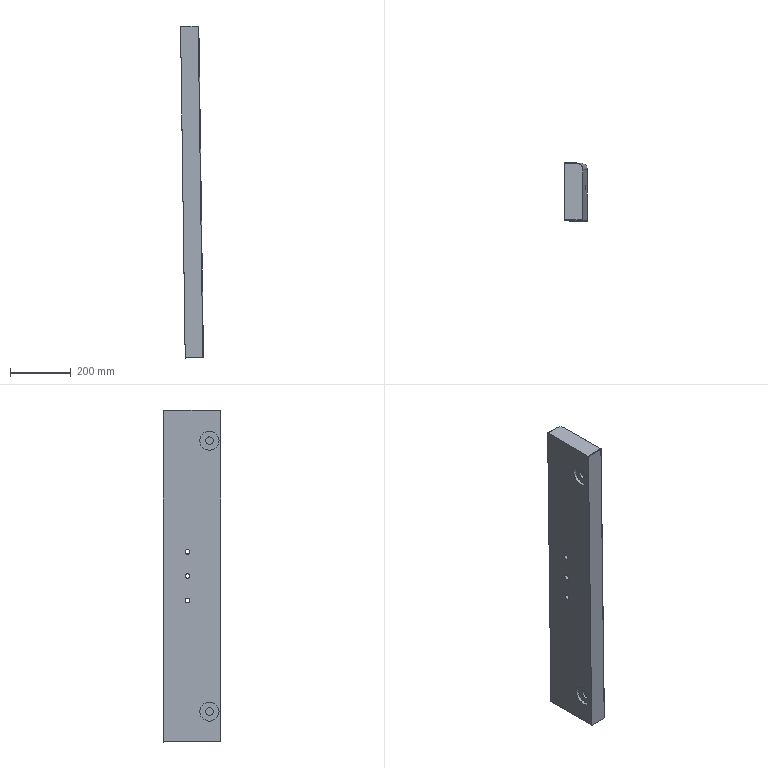Component | SolidWorks | DA-0220-Part9-4 | 1 solid | 35 faces | box 75.25 x 189.52 x 1090.68 mm | volume 12201627 mm3 | cylinder 22 | plane 10 | torus 2 | sphere 1 | commonest cylinder face diameters 4 x7 16 x6 25 x4 63 x4 40 x1
build123d program:
from build123d import *

# Parameters (mm, degrees)
SKETCH1_2_W                    = 60
SKETCH1_2_H                    = 189.5
BOSS_EXTRUDE1_DEPTH            = 545
FILLET1_R                      = 20
FILLET2_R                      = 2
SKETCH1_3_R                    = 8
CUT_EXTRUDE1_DEPTH             = 581.117
SKETCH1_R                      = 31.5
BUSHINGFLANGECOUNTERBORE_DEPTH = 8.5
SKETCH2_R                      = 12.5
GUIDESHAFTSEAT_DEPTH           = 16


with BuildPart() as part:
    # Sketch1_2 → Boss-Extrude1 (new, symmetric)
    with BuildSketch(Plane.XY):
        with Locations((30, 94.75)):
            Rectangle(SKETCH1_2_W, SKETCH1_2_H)
    extrude(amount=BOSS_EXTRUDE1_DEPTH, both=True)

    # Fillet1
    fillet1_edges = [part.edges().sort_by_distance(p)[0] for p in [
        (60, 189.5, 0),
    ]]
    fillet(fillet1_edges, radius=FILLET1_R)

    # Fillet2
    fillet2_edges = [part.edges().sort_by_distance(p)[0] for p in [
        (20, 189.5, -545),
        (20, 189.5, 545),
        (54.142, 183.642, -545),
        (54.142, 183.642, 545),
        (30, 0, 545),
        (0, 94.75, -545),
        (60, 84.75, -545),
        (60, 84.75, 545),
        (60, 0, 0),
    ]]
    fillet(fillet2_edges, radius=FILLET2_R)

    # Sketch1_3 → Cut-Extrude1 (cut, through all)
    with BuildSketch(Plane(origin=(60, 0, 0), x_dir=(0, 0, -1), z_dir=(1, 0, 0))):
        with Locations(Location((80, 109.5, 0), (0, 0, 90))):
            Circle(SKETCH1_3_R)
        with Locations(Location((0, 109.5, 0), (0, 0, 90))):
            Circle(SKETCH1_3_R)
        with Locations(Location((-80, 109.5, 0), (0, 0, 90))):
            Circle(SKETCH1_3_R)
    extrude(amount=-CUT_EXTRUDE1_DEPTH, mode=Mode.SUBTRACT)

    # Sketch1 → BushingFlangeCounterbore (cut)
    with BuildSketch(Plane.ZY):
        with Locations(Location((445, 37.5, 0), (0, 0, 270))):
            Circle(SKETCH1_R)
        with Locations(Location((-445, 37.5, 0), (0, 0, 270))):
            Circle(SKETCH1_R)
    extrude(amount=-BUSHINGFLANGECOUNTERBORE_DEPTH, mode=Mode.SUBTRACT)

    # Sketch2 → GuideShaftSeat (cut)
    with BuildSketch(Plane.ZY):
        with Locations(Location((445, 37.5, 0), (0, 0, 270))):
            Circle(SKETCH2_R)
        with Locations(Location((-445, 37.5, 0), (0, 0, 270))):
            Circle(SKETCH2_R)
    extrude(amount=-GUIDESHAFTSEAT_DEPTH, mode=Mode.SUBTRACT)


solid = part.part

# Placed as in the assembly
solid = solid.moved(Location((1026.124, -203.138, 17.82), (0.0001615, -0.7995, 0.02315)))
STEP:
#1=CARTESIAN_POINT('',(41.272,-6.029,-16.808));
#2=VERTEX_POINT('',#1);
#3=CARTESIAN_POINT('',(41.273,-7.013,-16.808));
#4=VERTEX_POINT('',#3);
#5=CARTESIAN_POINT('',(41.272,-6.521,-16.808));
#6=DIRECTION('',(-0.9999,-0.000404,-0.01395));
#7=DIRECTION('',(0.000404,-1.,0.00000282));
#8=AXIS2_PLACEMENT_3D('',#5,#6,#7);
#9=CIRCLE('',#8,0.4921);
#10=EDGE_CURVE('',#2,#4,#9,.T.);
#11=ORIENTED_EDGE('',*,*,#10,.F.);
#12=CARTESIAN_POINT('',(40.977,-6.029,-16.812));
#13=VERTEX_POINT('',#12);
#14=CARTESIAN_POINT('',(41.272,-6.029,-16.808));
#15=DIRECTION('',(-0.9999,-0.000404,-0.01395));
#16=VECTOR('',#15,39.37);
#17=LINE('',#14,#16);
#18=EDGE_CURVE('',#2,#13,#17,.T.);
#19=ORIENTED_EDGE('',*,*,#18,.T.);
#20=CARTESIAN_POINT('',(40.977,-7.013,-16.812));
#21=VERTEX_POINT('',#20);
#22=CARTESIAN_POINT('',(40.977,-6.521,-16.812));
#23=DIRECTION('',(-0.9999,-0.000404,-0.01395));
#24=DIRECTION('',(0.000404,-1.,0.00000282));
#25=AXIS2_PLACEMENT_3D('',#22,#23,#24);
#26=CIRCLE('',#25,0.4921);
#27=EDGE_CURVE('',#13,#21,#26,.T.);
#28=ORIENTED_EDGE('',*,*,#27,.T.);
#29=CARTESIAN_POINT('',(41.273,-7.013,-16.808));
#30=DIRECTION('',(-0.9999,-0.000404,-0.01395));
#31=VECTOR('',#30,39.37);
#32=LINE('',#29,#31);
#33=EDGE_CURVE('',#4,#21,#32,.T.);
#34=ORIENTED_EDGE('',*,*,#33,.F.);
#35=EDGE_LOOP('',(#11,#19,#28,#34));
#36=FACE_OUTER_BOUND('',#35,.T.);
#37=CARTESIAN_POINT('',(41.272,-6.521,-16.808));
#38=DIRECTION('',(-0.9999,-0.000404,-0.01395));
#39=DIRECTION('',(0.000404,-1.,0.00000282));
#40=AXIS2_PLACEMENT_3D('',#37,#38,#39);
#41=CYLINDRICAL_SURFACE('',#40,0.4921);
#42=ADVANCED_FACE('',(#36),#41,.F.);
#43=CARTESIAN_POINT('',(40.783,-6.029,18.228));
#44=VERTEX_POINT('',#43);
#45=CARTESIAN_POINT('',(40.784,-7.013,18.228));
#46=VERTEX_POINT('',#45);
#47=CARTESIAN_POINT('',(40.783,-6.521,18.228));
#48=DIRECTION('',(-0.9999,-0.000404,-0.01395));
#49=DIRECTION('',(0.000404,-1.,0.00000282));
#50=AXIS2_PLACEMENT_3D('',#47,#48,#49);
#51=CIRCLE('',#50,0.4921);
#52=EDGE_CURVE('',#44,#46,#51,.T.);
#53=ORIENTED_EDGE('',*,*,#52,.F.);
#54=CARTESIAN_POINT('',(40.488,-6.029,18.224));
#55=VERTEX_POINT('',#54);
#56=CARTESIAN_POINT('',(40.783,-6.029,18.228));
#57=DIRECTION('',(-0.9999,-0.000404,-0.01395));
#58=VECTOR('',#57,39.37);
#59=LINE('',#56,#58);
#60=EDGE_CURVE('',#44,#55,#59,.T.);
#61=ORIENTED_EDGE('',*,*,#60,.T.);
#62=CARTESIAN_POINT('',(40.488,-7.013,18.224));
#63=VERTEX_POINT('',#62);
#64=CARTESIAN_POINT('',(40.488,-6.521,18.224));
#65=DIRECTION('',(-0.9999,-0.000404,-0.01395));
#66=DIRECTION('',(0.000404,-1.,0.00000282));
#67=AXIS2_PLACEMENT_3D('',#64,#65,#66);
#68=CIRCLE('',#67,0.4921);
#69=EDGE_CURVE('',#55,#63,#68,.T.);
#70=ORIENTED_EDGE('',*,*,#69,.T.);
#71=CARTESIAN_POINT('',(40.784,-7.013,18.228));
#72=DIRECTION('',(-0.9999,-0.000404,-0.01395));
#73=VECTOR('',#72,39.37);
#74=LINE('',#71,#73);
#75=EDGE_CURVE('',#46,#63,#74,.T.);
#76=ORIENTED_EDGE('',*,*,#75,.F.);
#77=EDGE_LOOP('',(#53,#61,#70,#76));
#78=FACE_OUTER_BOUND('',#77,.T.);
#79=CARTESIAN_POINT('',(40.783,-6.521,18.228));
#80=DIRECTION('',(-0.9999,-0.000404,-0.01395));
#81=DIRECTION('',(0.000404,-1.,0.00000282));
#82=AXIS2_PLACEMENT_3D('',#79,#80,#81);
#83=CYLINDRICAL_SURFACE('',#82,0.4921);
#84=ADVANCED_FACE('',(#78),#83,.F.);
#85=CARTESIAN_POINT('',(40.488,-5.281,18.224));
#86=VERTEX_POINT('',#85);
#87=CARTESIAN_POINT('',(40.489,-7.761,18.224));
#88=VERTEX_POINT('',#87);
#89=CARTESIAN_POINT('',(40.488,-6.521,18.224));
#90=DIRECTION('',(-0.9999,-0.000404,-0.01395));
#91=DIRECTION('',(0.000404,-1.,0.00000282));
#92=AXIS2_PLACEMENT_3D('',#89,#90,#91);
#93=CIRCLE('',#92,1.24);
#94=EDGE_CURVE('',#86,#88,#93,.T.);
#95=ORIENTED_EDGE('',*,*,#94,.F.);
#96=CARTESIAN_POINT('',(40.153,-5.281,18.22));
#97=VERTEX_POINT('',#96);
#98=CARTESIAN_POINT('',(40.488,-5.281,18.224));
#99=DIRECTION('',(-0.9999,-0.000404,-0.01395));
#100=VECTOR('',#99,39.37);
#101=LINE('',#98,#100);
#102=EDGE_CURVE('',#86,#97,#101,.T.);
#103=ORIENTED_EDGE('',*,*,#102,.T.);
#104=CARTESIAN_POINT('',(40.154,-7.761,18.22));
#105=VERTEX_POINT('',#104);
#106=CARTESIAN_POINT('',(40.154,-6.521,18.22));
#107=DIRECTION('',(-0.9999,-0.000404,-0.01395));
#108=DIRECTION('',(0.000404,-1.,0.00000282));
#109=AXIS2_PLACEMENT_3D('',#106,#107,#108);
#110=CIRCLE('',#109,1.24);
#111=EDGE_CURVE('',#97,#105,#110,.T.);
#112=ORIENTED_EDGE('',*,*,#111,.T.);
#113=CARTESIAN_POINT('',(40.489,-7.761,18.224));
#114=DIRECTION('',(-0.9999,-0.000404,-0.01395));
#115=VECTOR('',#114,39.37);
#116=LINE('',#113,#115);
#117=EDGE_CURVE('',#88,#105,#116,.T.);
#118=ORIENTED_EDGE('',*,*,#117,.F.);
#119=EDGE_LOOP('',(#95,#103,#112,#118));
#120=FACE_OUTER_BOUND('',#119,.T.);
#121=CARTESIAN_POINT('',(40.488,-6.521,18.224));
#122=DIRECTION('',(-0.9999,-0.000404,-0.01395));
#123=DIRECTION('',(0.000404,-1.,0.00000282));
#124=AXIS2_PLACEMENT_3D('',#121,#122,#123);
#125=CYLINDRICAL_SURFACE('',#124,1.24);
#126=ADVANCED_FACE('',(#120),#125,.F.);
#127=CARTESIAN_POINT('',(40.977,-5.281,-16.812));
#128=VERTEX_POINT('',#127);
#129=CARTESIAN_POINT('',(40.978,-7.761,-16.812));
#130=VERTEX_POINT('',#129);
#131=CARTESIAN_POINT('',(40.977,-6.521,-16.812));
#132=DIRECTION('',(-0.9999,-0.000404,-0.01395));
#133=DIRECTION('',(0.000404,-1.,0.00000282));
#134=AXIS2_PLACEMENT_3D('',#131,#132,#133);
#135=CIRCLE('',#134,1.24);
#136=EDGE_CURVE('',#128,#130,#135,.T.);
#137=ORIENTED_EDGE('',*,*,#136,.F.);
#138=CARTESIAN_POINT('',(40.642,-5.281,-16.816));
#139=VERTEX_POINT('',#138);
#140=CARTESIAN_POINT('',(40.977,-5.281,-16.812));
#141=DIRECTION('',(-0.9999,-0.000404,-0.01395));
#142=VECTOR('',#141,39.37);
#143=LINE('',#140,#142);
#144=EDGE_CURVE('',#128,#139,#143,.T.);
#145=ORIENTED_EDGE('',*,*,#144,.T.);
#146=CARTESIAN_POINT('',(40.643,-7.761,-16.816));
#147=VERTEX_POINT('',#146);
#148=CARTESIAN_POINT('',(40.642,-6.521,-16.816));
#149=DIRECTION('',(-0.9999,-0.000404,-0.01395));
#150=DIRECTION('',(0.000404,-1.,0.00000282));
#151=AXIS2_PLACEMENT_3D('',#148,#149,#150);
#152=CIRCLE('',#151,1.24);
#153=EDGE_CURVE('',#139,#147,#152,.T.);
#154=ORIENTED_EDGE('',*,*,#153,.T.);
#155=CARTESIAN_POINT('',(40.978,-7.761,-16.812));
#156=DIRECTION('',(-0.9999,-0.000404,-0.01395));
#157=VECTOR('',#156,39.37);
#158=LINE('',#155,#157);
#159=EDGE_CURVE('',#130,#147,#158,.T.);
#160=ORIENTED_EDGE('',*,*,#159,.F.);
#161=EDGE_LOOP('',(#137,#145,#154,#160));
#162=FACE_OUTER_BOUND('',#161,.T.);
#163=CARTESIAN_POINT('',(40.977,-6.521,-16.812));
#164=DIRECTION('',(-0.9999,-0.000404,-0.01395));
#165=DIRECTION('',(0.000404,-1.,0.00000282));
#166=AXIS2_PLACEMENT_3D('',#163,#164,#165);
#167=CYLINDRICAL_SURFACE('',#166,1.24);
#168=ADVANCED_FACE('',(#162),#167,.F.);
#169=CARTESIAN_POINT('',(40.353,-4.001,3.851));
#170=VERTEX_POINT('',#169);
#171=CARTESIAN_POINT('',(40.353,-3.372,3.851));
#172=VERTEX_POINT('',#171);
#173=CARTESIAN_POINT('',(40.353,-3.687,3.851));
#174=DIRECTION('',(0.9999,0.000404,0.01395));
#175=DIRECTION('',(0.000404,-1.,0.00000282));
#176=AXIS2_PLACEMENT_3D('',#173,#174,#175);
#177=CIRCLE('',#176,0.315);
#178=EDGE_CURVE('',#170,#172,#177,.T.);
#179=ORIENTED_EDGE('',*,*,#178,.F.);
#180=CARTESIAN_POINT('',(42.715,-4.001,3.884));
#181=VERTEX_POINT('',#180);
#182=CARTESIAN_POINT('',(40.353,-4.001,3.851));
#183=DIRECTION('',(0.9999,0.000404,0.01395));
#184=VECTOR('',#183,39.37);
#185=LINE('',#182,#184);
#186=EDGE_CURVE('',#170,#181,#185,.T.);
#187=ORIENTED_EDGE('',*,*,#186,.T.);
#188=CARTESIAN_POINT('',(42.715,-3.371,3.884));
#189=VERTEX_POINT('',#188);
#190=CARTESIAN_POINT('',(42.715,-3.686,3.884));
#191=DIRECTION('',(0.9999,0.000404,0.01395));
#192=DIRECTION('',(0.000404,-1.,0.00000282));
#193=AXIS2_PLACEMENT_3D('',#190,#191,#192);
#194=CIRCLE('',#193,0.315);
#195=EDGE_CURVE('',#181,#189,#194,.T.);
#196=ORIENTED_EDGE('',*,*,#195,.T.);
#197=CARTESIAN_POINT('',(40.353,-3.372,3.851));
#198=DIRECTION('',(0.9999,0.000404,0.01395));
#199=VECTOR('',#198,39.37);
#200=LINE('',#197,#199);
#201=EDGE_CURVE('',#172,#189,#200,.T.);
#202=ORIENTED_EDGE('',*,*,#201,.F.);
#203=EDGE_LOOP('',(#179,#187,#196,#202));
#204=FACE_OUTER_BOUND('',#203,.T.);
#205=CARTESIAN_POINT('',(40.353,-3.687,3.851));
#206=DIRECTION('',(0.9999,0.000404,0.01395));
#207=DIRECTION('',(-0.000404,1.,-0.00000282));
#208=AXIS2_PLACEMENT_3D('',#205,#206,#207);
#209=CYLINDRICAL_SURFACE('',#208,0.315);
#210=ADVANCED_FACE('',(#204),#209,.F.);
#211=CARTESIAN_POINT('',(40.397,-4.001,0.7016));
#212=VERTEX_POINT('',#211);
#213=CARTESIAN_POINT('',(40.397,-3.372,0.7016));
#214=VERTEX_POINT('',#213);
#215=CARTESIAN_POINT('',(40.397,-3.687,0.7016));
#216=DIRECTION('',(0.9999,0.000404,0.01395));
#217=DIRECTION('',(0.000404,-1.,0.00000282));
#218=AXIS2_PLACEMENT_3D('',#215,#216,#217);
#219=CIRCLE('',#218,0.315);
#220=EDGE_CURVE('',#212,#214,#219,.T.);
#221=ORIENTED_EDGE('',*,*,#220,.F.);
#222=CARTESIAN_POINT('',(42.759,-4.001,0.7345));
#223=VERTEX_POINT('',#222);
#224=CARTESIAN_POINT('',(40.397,-4.001,0.7016));
#225=DIRECTION('',(0.9999,0.000404,0.01395));
#226=VECTOR('',#225,39.37);
#227=LINE('',#224,#226);
#228=EDGE_CURVE('',#212,#223,#227,.T.);
#229=ORIENTED_EDGE('',*,*,#228,.T.);
#230=CARTESIAN_POINT('',(42.759,-3.371,0.7345));
#231=VERTEX_POINT('',#230);
#232=CARTESIAN_POINT('',(42.759,-3.686,0.7345));
#233=DIRECTION('',(0.9999,0.000404,0.01395));
#234=DIRECTION('',(0.000404,-1.,0.00000282));
#235=AXIS2_PLACEMENT_3D('',#232,#233,#234);
#236=CIRCLE('',#235,0.315);
#237=EDGE_CURVE('',#223,#231,#236,.T.);
#238=ORIENTED_EDGE('',*,*,#237,.T.);
#239=CARTESIAN_POINT('',(40.397,-3.372,0.7016));
#240=DIRECTION('',(0.9999,0.000404,0.01395));
#241=VECTOR('',#240,39.37);
#242=LINE('',#239,#241);
#243=EDGE_CURVE('',#214,#231,#242,.T.);
#244=ORIENTED_EDGE('',*,*,#243,.F.);
#245=EDGE_LOOP('',(#221,#229,#238,#244));
#246=FACE_OUTER_BOUND('',#245,.T.);
#247=CARTESIAN_POINT('',(40.397,-3.687,0.7016));
#248=DIRECTION('',(0.9999,0.000404,0.01395));
#249=DIRECTION('',(-0.000404,1.,-0.00000282));
#250=AXIS2_PLACEMENT_3D('',#247,#248,#249);
#251=CYLINDRICAL_SURFACE('',#250,0.315);
#252=ADVANCED_FACE('',(#246),#251,.F.);
#253=CARTESIAN_POINT('',(40.441,-4.001,-2.448));
#254=VERTEX_POINT('',#253);
#255=CARTESIAN_POINT('',(40.441,-3.372,-2.448));
#256=VERTEX_POINT('',#255);
#257=CARTESIAN_POINT('',(40.441,-3.687,-2.448));
#258=DIRECTION('',(0.9999,0.000404,0.01395));
#259=DIRECTION('',(0.000404,-1.,0.00000282));
#260=AXIS2_PLACEMENT_3D('',#257,#258,#259);
#261=CIRCLE('',#260,0.315);
#262=EDGE_CURVE('',#254,#256,#261,.T.);
#263=ORIENTED_EDGE('',*,*,#262,.F.);
#264=CARTESIAN_POINT('',(42.803,-4.001,-2.415));
#265=VERTEX_POINT('',#264);
#266=CARTESIAN_POINT('',(40.441,-4.001,-2.448));
#267=DIRECTION('',(0.9999,0.000404,0.01395));
#268=VECTOR('',#267,39.37);
#269=LINE('',#266,#268);
#270=EDGE_CURVE('',#254,#265,#269,.T.);
#271=ORIENTED_EDGE('',*,*,#270,.T.);
#272=CARTESIAN_POINT('',(42.803,-3.371,-2.415));
#273=VERTEX_POINT('',#272);
#274=CARTESIAN_POINT('',(42.803,-3.686,-2.415));
#275=DIRECTION('',(0.9999,0.000404,0.01395));
#276=DIRECTION('',(0.000404,-1.,0.00000282));
#277=AXIS2_PLACEMENT_3D('',#274,#275,#276);
#278=CIRCLE('',#277,0.315);
#279=EDGE_CURVE('',#265,#273,#278,.T.);
#280=ORIENTED_EDGE('',*,*,#279,.T.);
#281=CARTESIAN_POINT('',(40.441,-3.372,-2.448));
#282=DIRECTION('',(0.9999,0.000404,0.01395));
#283=VECTOR('',#282,39.37);
#284=LINE('',#281,#283);
#285=EDGE_CURVE('',#256,#273,#284,.T.);
#286=ORIENTED_EDGE('',*,*,#285,.F.);
#287=EDGE_LOOP('',(#263,#271,#280,#286));
#288=FACE_OUTER_BOUND('',#287,.T.);
#289=CARTESIAN_POINT('',(40.441,-3.687,-2.448));
#290=DIRECTION('',(0.9999,0.000404,0.01395));
#291=DIRECTION('',(-0.000404,1.,-0.00000282));
#292=AXIS2_PLACEMENT_3D('',#289,#290,#291);
#293=CYLINDRICAL_SURFACE('',#292,0.315);
#294=ADVANCED_FACE('',(#288),#293,.F.);
#295=CARTESIAN_POINT('',(40.1,-7.998,22.077));
#296=VERTEX_POINT('',#295);
#297=CARTESIAN_POINT('',(40.697,-7.997,-20.674));
#298=VERTEX_POINT('',#297);
#299=CARTESIAN_POINT('',(40.099,-7.998,22.156));
#300=DIRECTION('',(0.01395,0.00000282,-0.9999));
#301=VECTOR('',#300,39.37);
#302=LINE('',#299,#301);
#303=EDGE_CURVE('',#296,#298,#302,.T.);
#304=ORIENTED_EDGE('',*,*,#303,.T.);
#305=CARTESIAN_POINT('',(40.777,-7.997,-20.752));
#306=VERTEX_POINT('',#305);
#307=CARTESIAN_POINT('',(40.776,-7.997,-20.673));
#308=DIRECTION('',(0.000404,-1.,0.00000282));
#309=DIRECTION('',(-0.9999,-0.000404,-0.01395));
#310=AXIS2_PLACEMENT_3D('',#307,#308,#309);
#311=CIRCLE('',#310,0.07874);
#312=EDGE_CURVE('',#298,#306,#311,.T.);
#313=ORIENTED_EDGE('',*,*,#312,.T.);
#314=CARTESIAN_POINT('',(42.981,-7.997,-20.721));
#315=VERTEX_POINT('',#314);
#316=CARTESIAN_POINT('',(43.06,-7.997,-20.72));
#317=DIRECTION('',(0.9999,0.000404,0.01395));
#318=VECTOR('',#317,39.37);
#319=LINE('',#316,#318);
#320=EDGE_CURVE('',#306,#315,#319,.T.);
#321=ORIENTED_EDGE('',*,*,#320,.T.);
#322=CARTESIAN_POINT('',(42.384,-7.997,22.109));
#323=VERTEX_POINT('',#322);
#324=CARTESIAN_POINT('',(42.382,-7.997,22.188));
#325=DIRECTION('',(-0.01395,-0.00000282,0.9999));
#326=VECTOR('',#325,39.37);
#327=LINE('',#324,#326);
#328=EDGE_CURVE('',#315,#323,#327,.T.);
#329=ORIENTED_EDGE('',*,*,#328,.T.);
#330=CARTESIAN_POINT('',(42.462,-7.997,22.11));
#331=DIRECTION('',(-0.9999,-0.000404,-0.01395));
#332=VECTOR('',#331,39.37);
#333=LINE('',#330,#332);
#334=EDGE_CURVE('',#323,#296,#333,.T.);
#335=ORIENTED_EDGE('',*,*,#334,.T.);
#336=EDGE_LOOP('',(#304,#313,#321,#329,#335));
#337=FACE_OUTER_BOUND('',#336,.T.);
#338=CARTESIAN_POINT('',(42.461,-7.997,22.189));
#339=DIRECTION('',(-0.000404,1.,-0.00000282));
#340=DIRECTION('',(-0.9999,-0.000404,-0.01395));
#341=AXIS2_PLACEMENT_3D('',#338,#339,#340);
#342=PLANE('',#341);
#343=ADVANCED_FACE('',(#337),#342,.F.);
#344=CARTESIAN_POINT('',(42.715,-3.686,3.884));
#345=DIRECTION('',(0.9999,0.000404,0.01395));
#346=DIRECTION('',(0.000404,-1.,0.00000282));
#347=AXIS2_PLACEMENT_3D('',#344,#345,#346);
#348=CIRCLE('',#347,0.315);
#349=EDGE_CURVE('',#189,#181,#348,.T.);
#350=ORIENTED_EDGE('',*,*,#349,.F.);
#351=ORIENTED_EDGE('',*,*,#195,.F.);
#352=EDGE_LOOP('',(#350,#351));
#353=FACE_BOUND('',#352,.T.);
#354=CARTESIAN_POINT('',(42.759,-3.686,0.7345));
#355=DIRECTION('',(0.9999,0.000404,0.01395));
#356=DIRECTION('',(0.000404,-1.,0.00000282));
#357=AXIS2_PLACEMENT_3D('',#354,#355,#356);
#358=CIRCLE('',#357,0.315);
#359=EDGE_CURVE('',#231,#223,#358,.T.);
#360=ORIENTED_EDGE('',*,*,#359,.F.);
#361=ORIENTED_EDGE('',*,*,#237,.F.);
#362=EDGE_LOOP('',(#360,#361));
#363=FACE_BOUND('',#362,.T.);
#364=CARTESIAN_POINT('',(42.803,-3.686,-2.415));
#365=DIRECTION('',(0.9999,0.000404,0.01395));
#366=DIRECTION('',(0.000404,-1.,0.00000282));
#367=AXIS2_PLACEMENT_3D('',#364,#365,#366);
#368=CIRCLE('',#367,0.315);
#369=EDGE_CURVE('',#273,#265,#368,.T.);
#370=ORIENTED_EDGE('',*,*,#369,.F.);
#371=ORIENTED_EDGE('',*,*,#279,.F.);
#372=EDGE_LOOP('',(#370,#371));
#373=FACE_BOUND('',#372,.T.);
#374=CARTESIAN_POINT('',(42.462,-7.918,22.11));
#375=VERTEX_POINT('',#374);
#376=CARTESIAN_POINT('',(43.059,-7.918,-20.641));
#377=VERTEX_POINT('',#376);
#378=CARTESIAN_POINT('',(42.461,-7.918,22.189));
#379=DIRECTION('',(0.01395,0.00000282,-0.9999));
#380=VECTOR('',#379,39.37);
#381=LINE('',#378,#380);
#382=EDGE_CURVE('',#375,#377,#381,.T.);
#383=ORIENTED_EDGE('',*,*,#382,.T.);
#384=CARTESIAN_POINT('',(43.056,-1.323,-20.641));
#385=VERTEX_POINT('',#384);
#386=CARTESIAN_POINT('',(43.056,-1.323,-20.641));
#387=DIRECTION('',(-0.000404,1.,-0.00000282));
#388=VECTOR('',#387,39.37);
#389=LINE('',#386,#388);
#390=EDGE_CURVE('',#377,#385,#389,.T.);
#391=ORIENTED_EDGE('',*,*,#390,.T.);
#392=CARTESIAN_POINT('',(42.46,-1.323,22.11));
#393=VERTEX_POINT('',#392);
#394=CARTESIAN_POINT('',(42.458,-1.323,22.189));
#395=DIRECTION('',(-0.01395,-0.00000282,0.9999));
#396=VECTOR('',#395,39.37);
#397=LINE('',#394,#396);
#398=EDGE_CURVE('',#385,#393,#397,.T.);
#399=ORIENTED_EDGE('',*,*,#398,.T.);
#400=CARTESIAN_POINT('',(42.459,-0.536,22.11));
#401=DIRECTION('',(0.000404,-1.,0.00000282));
#402=VECTOR('',#401,39.37);
#403=LINE('',#400,#402);
#404=EDGE_CURVE('',#393,#375,#403,.T.);
#405=ORIENTED_EDGE('',*,*,#404,.T.);
#406=EDGE_LOOP('',(#383,#391,#399,#405));
#407=FACE_OUTER_BOUND('',#406,.T.);
#408=CARTESIAN_POINT('',(42.458,-0.536,22.189));
#409=DIRECTION('',(-0.9999,-0.000404,-0.01395));
#410=DIRECTION('',(0.000404,-1.,0.00000282));
#411=AXIS2_PLACEMENT_3D('',#408,#409,#410);
#412=PLANE('',#411);
#413=ADVANCED_FACE('',(#353,#363,#373,#407),#412,.F.);
#414=CARTESIAN_POINT('',(41.672,-0.5363,22.099));
#415=VERTEX_POINT('',#414);
#416=CARTESIAN_POINT('',(42.269,-0.5362,-20.652));
#417=VERTEX_POINT('',#416);
#418=CARTESIAN_POINT('',(41.671,-0.5363,22.178));
#419=DIRECTION('',(0.01395,0.00000282,-0.9999));
#420=VECTOR('',#419,39.37);
#421=LINE('',#418,#420);
#422=EDGE_CURVE('',#415,#417,#421,.T.);
#423=ORIENTED_EDGE('',*,*,#422,.T.);
#424=CARTESIAN_POINT('',(40.694,-0.5369,-20.674));
#425=VERTEX_POINT('',#424);
#426=CARTESIAN_POINT('',(40.694,-0.5369,-20.674));
#427=DIRECTION('',(-0.9999,-0.000404,-0.01395));
#428=VECTOR('',#427,39.37);
#429=LINE('',#426,#428);
#430=EDGE_CURVE('',#417,#425,#429,.T.);
#431=ORIENTED_EDGE('',*,*,#430,.T.);
#432=CARTESIAN_POINT('',(40.097,-0.537,22.077));
#433=VERTEX_POINT('',#432);
#434=CARTESIAN_POINT('',(40.096,-0.537,22.156));
#435=DIRECTION('',(0.01395,0.00000282,-0.9999));
#436=VECTOR('',#435,39.37);
#437=LINE('',#434,#436);
#438=EDGE_CURVE('',#433,#425,#437,.T.);
#439=ORIENTED_EDGE('',*,*,#438,.F.);
#440=CARTESIAN_POINT('',(40.097,-0.537,22.077));
#441=DIRECTION('',(0.9999,0.000404,0.01395));
#442=VECTOR('',#441,39.37);
#443=LINE('',#440,#442);
#444=EDGE_CURVE('',#433,#415,#443,.T.);
#445=ORIENTED_EDGE('',*,*,#444,.T.);
#446=EDGE_LOOP('',(#423,#431,#439,#445));
#447=FACE_OUTER_BOUND('',#446,.T.);
#448=CARTESIAN_POINT('',(40.096,-0.537,22.156));
#449=DIRECTION('',(0.000404,-1.,0.00000282));
#450=DIRECTION('',(0.01395,0.00000282,-0.9999));
#451=AXIS2_PLACEMENT_3D('',#448,#449,#450);
#452=PLANE('',#451);
#453=ADVANCED_FACE('',(#447),#452,.F.);
#454=CARTESIAN_POINT('',(40.154,-6.521,18.22));
#455=DIRECTION('',(-0.9999,-0.000404,-0.01395));
#456=DIRECTION('',(0.000404,-1.,0.00000282));
#457=AXIS2_PLACEMENT_3D('',#454,#455,#456);
#458=CIRCLE('',#457,1.24);
#459=EDGE_CURVE('',#105,#97,#458,.T.);
#460=ORIENTED_EDGE('',*,*,#459,.F.);
#461=ORIENTED_EDGE('',*,*,#111,.F.);
#462=EDGE_LOOP('',(#460,#461));
#463=FACE_BOUND('',#462,.T.);
#464=CARTESIAN_POINT('',(40.642,-6.521,-16.816));
#465=DIRECTION('',(-0.9999,-0.000404,-0.01395));
#466=DIRECTION('',(0.000404,-1.,0.00000282));
#467=AXIS2_PLACEMENT_3D('',#464,#465,#466);
#468=CIRCLE('',#467,1.24);
#469=EDGE_CURVE('',#147,#139,#468,.T.);
#470=ORIENTED_EDGE('',*,*,#469,.F.);
#471=ORIENTED_EDGE('',*,*,#153,.F.);
#472=EDGE_LOOP('',(#470,#471));
#473=FACE_BOUND('',#472,.T.);
#474=CARTESIAN_POINT('',(40.353,-3.687,3.851));
#475=DIRECTION('',(0.9999,0.000404,0.01395));
#476=DIRECTION('',(0.000404,-1.,0.00000282));
#477=AXIS2_PLACEMENT_3D('',#474,#475,#476);
#478=CIRCLE('',#477,0.315);
#479=EDGE_CURVE('',#172,#170,#478,.T.);
#480=ORIENTED_EDGE('',*,*,#479,.T.);
#481=ORIENTED_EDGE('',*,*,#178,.T.);
#482=EDGE_LOOP('',(#480,#481));
#483=FACE_BOUND('',#482,.T.);
#484=CARTESIAN_POINT('',(40.397,-3.687,0.7016));
#485=DIRECTION('',(0.9999,0.000404,0.01395));
#486=DIRECTION('',(0.000404,-1.,0.00000282));
#487=AXIS2_PLACEMENT_3D('',#484,#485,#486);
#488=CIRCLE('',#487,0.315);
#489=EDGE_CURVE('',#214,#212,#488,.T.);
#490=ORIENTED_EDGE('',*,*,#489,.T.);
#491=ORIENTED_EDGE('',*,*,#220,.T.);
#492=EDGE_LOOP('',(#490,#491));
#493=FACE_BOUND('',#492,.T.);
#494=CARTESIAN_POINT('',(40.441,-3.687,-2.448));
#495=DIRECTION('',(0.9999,0.000404,0.01395));
#496=DIRECTION('',(0.000404,-1.,0.00000282));
#497=AXIS2_PLACEMENT_3D('',#494,#495,#496);
#498=CIRCLE('',#497,0.315);
#499=EDGE_CURVE('',#256,#254,#498,.T.);
#500=ORIENTED_EDGE('',*,*,#499,.T.);
#501=ORIENTED_EDGE('',*,*,#262,.T.);
#502=EDGE_LOOP('',(#500,#501));
#503=FACE_BOUND('',#502,.T.);
#504=CARTESIAN_POINT('',(40.096,-0.6157,22.156));
#505=VERTEX_POINT('',#504);
#506=CARTESIAN_POINT('',(40.099,-7.919,22.156));
#507=VERTEX_POINT('',#506);
#508=CARTESIAN_POINT('',(40.099,-7.998,22.156));
#509=DIRECTION('',(0.000404,-1.,0.00000282));
#510=VECTOR('',#509,39.37);
#511=LINE('',#508,#510);
#512=EDGE_CURVE('',#505,#507,#511,.T.);
#513=ORIENTED_EDGE('',*,*,#512,.F.);
#514=CARTESIAN_POINT('',(40.097,-0.6157,22.077));
#515=DIRECTION('',(-0.9999,-0.000404,-0.01395));
#516=DIRECTION('',(-0.000404,1.,-0.00000282));
#517=AXIS2_PLACEMENT_3D('',#514,#515,#516);
#518=CIRCLE('',#517,0.07874);
#519=EDGE_CURVE('',#505,#433,#518,.T.);
#520=ORIENTED_EDGE('',*,*,#519,.T.);
#521=ORIENTED_EDGE('',*,*,#438,.T.);
#522=CARTESIAN_POINT('',(40.697,-7.997,-20.674));
#523=DIRECTION('',(0.000404,-1.,0.00000282));
#524=VECTOR('',#523,39.37);
#525=LINE('',#522,#524);
#526=EDGE_CURVE('',#425,#298,#525,.T.);
#527=ORIENTED_EDGE('',*,*,#526,.T.);
#528=ORIENTED_EDGE('',*,*,#303,.F.);
#529=CARTESIAN_POINT('',(40.1,-7.919,22.077));
#530=DIRECTION('',(-0.9999,-0.000404,-0.01395));
#531=DIRECTION('',(-0.000404,1.,-0.00000282));
#532=AXIS2_PLACEMENT_3D('',#529,#530,#531);
#533=CIRCLE('',#532,0.07874);
#534=EDGE_CURVE('',#296,#507,#533,.T.);
#535=ORIENTED_EDGE('',*,*,#534,.T.);
#536=EDGE_LOOP('',(#513,#520,#521,#527,#528,#535));
#537=FACE_OUTER_BOUND('',#536,.T.);
#538=CARTESIAN_POINT('',(40.099,-7.998,22.156));
#539=DIRECTION('',(0.9999,0.000404,0.01395));
#540=DIRECTION('',(-0.000404,1.,-0.00000282));
#541=AXIS2_PLACEMENT_3D('',#538,#539,#540);
#542=PLANE('',#541);
#543=ADVANCED_FACE('',(#463,#473,#483,#493,#503,#537),#542,.F.);
#544=CARTESIAN_POINT('',(42.38,-1.323,22.188));
#545=VERTEX_POINT('',#544);
#546=CARTESIAN_POINT('',(41.671,-0.6151,22.178));
#547=VERTEX_POINT('',#546);
#548=CARTESIAN_POINT('',(41.671,-1.324,22.178));
#549=DIRECTION('',(-0.01395,-0.00000282,0.9999));
#550=DIRECTION('',(-0.9999,-0.000404,-0.01395));
#551=AXIS2_PLACEMENT_3D('',#548,#549,#550);
#552=CIRCLE('',#551,0.7087);
#553=EDGE_CURVE('',#545,#547,#552,.T.);
#554=ORIENTED_EDGE('',*,*,#553,.T.);
#555=CARTESIAN_POINT('',(40.096,-0.6157,22.156));
#556=DIRECTION('',(-0.9999,-0.000404,-0.01395));
#557=VECTOR('',#556,39.37);
#558=LINE('',#555,#557);
#559=EDGE_CURVE('',#547,#505,#558,.T.);
#560=ORIENTED_EDGE('',*,*,#559,.T.);
#561=ORIENTED_EDGE('',*,*,#512,.T.);
#562=CARTESIAN_POINT('',(42.382,-7.918,22.188));
#563=VERTEX_POINT('',#562);
#564=CARTESIAN_POINT('',(40.099,-7.919,22.156));
#565=DIRECTION('',(0.9999,0.000404,0.01395));
#566=VECTOR('',#565,39.37);
#567=LINE('',#564,#566);
#568=EDGE_CURVE('',#507,#563,#567,.T.);
#569=ORIENTED_EDGE('',*,*,#568,.T.);
#570=CARTESIAN_POINT('',(42.382,-7.997,22.188));
#571=DIRECTION('',(-0.000404,1.,-0.00000282));
#572=VECTOR('',#571,39.37);
#573=LINE('',#570,#572);
#574=EDGE_CURVE('',#563,#545,#573,.T.);
#575=ORIENTED_EDGE('',*,*,#574,.T.);
#576=EDGE_LOOP('',(#554,#560,#561,#569,#575));
#577=FACE_OUTER_BOUND('',#576,.T.);
#578=CARTESIAN_POINT('',(40.099,-7.998,22.156));
#579=DIRECTION('',(0.01395,0.00000282,-0.9999));
#580=DIRECTION('',(-0.9999,-0.000404,-0.01395));
#581=AXIS2_PLACEMENT_3D('',#578,#579,#580);
#582=PLANE('',#581);
#583=ADVANCED_FACE('',(#577),#582,.F.);
#584=ORIENTED_EDGE('',*,*,#320,.F.);
#585=CARTESIAN_POINT('',(40.774,-0.6156,-20.752));
#586=VERTEX_POINT('',#585);
#587=CARTESIAN_POINT('',(40.774,-0.5368,-20.752));
#588=DIRECTION('',(-0.000404,1.,-0.00000282));
#589=VECTOR('',#588,39.37);
#590=LINE('',#587,#589);
#591=EDGE_CURVE('',#306,#586,#590,.T.);
#592=ORIENTED_EDGE('',*,*,#591,.T.);
#593=CARTESIAN_POINT('',(42.27,-0.615,-20.731));
#594=VERTEX_POINT('',#593);
#595=CARTESIAN_POINT('',(42.27,-0.615,-20.731));
#596=DIRECTION('',(0.9999,0.000404,0.01395));
#597=VECTOR('',#596,39.37);
#598=LINE('',#595,#597);
#599=EDGE_CURVE('',#586,#594,#598,.T.);
#600=ORIENTED_EDGE('',*,*,#599,.T.);
#601=CARTESIAN_POINT('',(42.979,-1.323,-20.721));
#602=VERTEX_POINT('',#601);
#603=CARTESIAN_POINT('',(42.27,-1.324,-20.731));
#604=DIRECTION('',(0.01395,0.00000282,-0.9999));
#605=DIRECTION('',(-0.9999,-0.000404,-0.01395));
#606=AXIS2_PLACEMENT_3D('',#603,#604,#605);
#607=CIRCLE('',#606,0.7087);
#608=EDGE_CURVE('',#594,#602,#607,.T.);
#609=ORIENTED_EDGE('',*,*,#608,.T.);
#610=CARTESIAN_POINT('',(42.981,-7.997,-20.721));
#611=DIRECTION('',(0.000404,-1.,0.00000282));
#612=VECTOR('',#611,39.37);
#613=LINE('',#610,#612);
#614=EDGE_CURVE('',#602,#315,#613,.T.);
#615=ORIENTED_EDGE('',*,*,#614,.T.);
#616=EDGE_LOOP('',(#584,#592,#600,#609,#615));
#617=FACE_OUTER_BOUND('',#616,.T.);
#618=CARTESIAN_POINT('',(40.698,-7.997,-20.753));
#619=DIRECTION('',(0.01395,0.00000282,-0.9999));
#620=DIRECTION('',(-0.9999,-0.000404,-0.01395));
#621=AXIS2_PLACEMENT_3D('',#618,#619,#620);
#622=PLANE('',#621);
#623=ADVANCED_FACE('',(#617),#622,.T.);
#624=ORIENTED_EDGE('',*,*,#398,.F.);
#625=CARTESIAN_POINT('',(42.269,-1.324,-20.652));
#626=DIRECTION('',(-0.01395,-0.00000282,0.9999));
#627=DIRECTION('',(-0.9999,-0.000404,-0.01395));
#628=AXIS2_PLACEMENT_3D('',#625,#626,#627);
#629=CIRCLE('',#628,0.7874);
#630=EDGE_CURVE('',#385,#417,#629,.T.);
#631=ORIENTED_EDGE('',*,*,#630,.T.);
#632=ORIENTED_EDGE('',*,*,#422,.F.);
#633=CARTESIAN_POINT('',(41.672,-1.324,22.099));
#634=DIRECTION('',(0.01395,0.00000282,-0.9999));
#635=DIRECTION('',(-0.9999,-0.000404,-0.01395));
#636=AXIS2_PLACEMENT_3D('',#633,#634,#635);
#637=CIRCLE('',#636,0.7874);
#638=EDGE_CURVE('',#415,#393,#637,.T.);
#639=ORIENTED_EDGE('',*,*,#638,.T.);
#640=EDGE_LOOP('',(#624,#631,#632,#639));
#641=FACE_OUTER_BOUND('',#640,.T.);
#642=CARTESIAN_POINT('',(41.671,-1.324,22.178));
#643=DIRECTION('',(0.01395,0.00000282,-0.9999));
#644=DIRECTION('',(-0.9999,-0.000404,-0.01395));
#645=AXIS2_PLACEMENT_3D('',#642,#643,#644);
#646=CYLINDRICAL_SURFACE('',#645,0.7874);
#647=ADVANCED_FACE('',(#641),#646,.T.);
#648=ORIENTED_EDGE('',*,*,#519,.F.);
#649=ORIENTED_EDGE('',*,*,#559,.F.);
#650=CARTESIAN_POINT('',(41.672,-0.6151,22.099));
#651=DIRECTION('',(0.9999,0.000404,0.01395));
#652=DIRECTION('',(0.01395,0.00000282,-0.9999));
#653=AXIS2_PLACEMENT_3D('',#650,#651,#652);
#654=CIRCLE('',#653,0.07874);
#655=EDGE_CURVE('',#415,#547,#654,.T.);
#656=ORIENTED_EDGE('',*,*,#655,.F.);
#657=ORIENTED_EDGE('',*,*,#444,.F.);
#658=EDGE_LOOP('',(#648,#649,#656,#657));
#659=FACE_OUTER_BOUND('',#658,.T.);
#660=CARTESIAN_POINT('',(40.097,-0.6157,22.077));
#661=DIRECTION('',(-0.9999,-0.000404,-0.01395));
#662=DIRECTION('',(-0.01395,-0.00000282,0.9999));
#663=AXIS2_PLACEMENT_3D('',#660,#661,#662);
#664=CYLINDRICAL_SURFACE('',#663,0.07874);
#665=ADVANCED_FACE('',(#659),#664,.T.);
#666=ORIENTED_EDGE('',*,*,#655,.T.);
#667=ORIENTED_EDGE('',*,*,#553,.F.);
#668=CARTESIAN_POINT('',(42.381,-1.323,22.109));
#669=DIRECTION('',(0.000404,-1.,0.00000282));
#670=DIRECTION('',(0.01395,0.00000282,-0.9999));
#671=AXIS2_PLACEMENT_3D('',#668,#669,#670);
#672=CIRCLE('',#671,0.07874);
#673=EDGE_CURVE('',#393,#545,#672,.T.);
#674=ORIENTED_EDGE('',*,*,#673,.F.);
#675=ORIENTED_EDGE('',*,*,#638,.F.);
#676=EDGE_LOOP('',(#666,#667,#674,#675));
#677=FACE_OUTER_BOUND('',#676,.T.);
#678=CARTESIAN_POINT('',(41.672,-1.324,22.099));
#679=DIRECTION('',(0.01395,0.00000282,-0.9999));
#680=DIRECTION('',(-0.9999,-0.000404,-0.01395));
#681=AXIS2_PLACEMENT_3D('',#678,#679,#680);
#682=TOROIDAL_SURFACE('',#681,0.7087,0.07874);
#683=ADVANCED_FACE('',(#677),#682,.T.);
#684=ORIENTED_EDGE('',*,*,#534,.F.);
#685=ORIENTED_EDGE('',*,*,#334,.F.);
#686=CARTESIAN_POINT('',(42.383,-7.918,22.109));
#687=DIRECTION('',(0.9999,0.000404,0.01395));
#688=DIRECTION('',(0.01395,0.00000282,-0.9999));
#689=AXIS2_PLACEMENT_3D('',#686,#687,#688);
#690=CIRCLE('',#689,0.07874);
#691=EDGE_CURVE('',#563,#323,#690,.T.);
#692=ORIENTED_EDGE('',*,*,#691,.F.);
#693=ORIENTED_EDGE('',*,*,#568,.F.);
#694=EDGE_LOOP('',(#684,#685,#692,#693));
#695=FACE_OUTER_BOUND('',#694,.T.);
#696=CARTESIAN_POINT('',(40.1,-7.919,22.077));
#697=DIRECTION('',(0.9999,0.000404,0.01395));
#698=DIRECTION('',(-0.000404,1.,-0.00000282));
#699=AXIS2_PLACEMENT_3D('',#696,#697,#698);
#700=CYLINDRICAL_SURFACE('',#699,0.07874);
#701=ADVANCED_FACE('',(#695),#700,.T.);
#702=ORIENTED_EDGE('',*,*,#673,.T.);
#703=ORIENTED_EDGE('',*,*,#574,.F.);
#704=CARTESIAN_POINT('',(42.383,-7.918,22.109));
#705=DIRECTION('',(0.000404,-1.,0.00000282));
#706=DIRECTION('',(0.01395,0.00000282,-0.9999));
#707=AXIS2_PLACEMENT_3D('',#704,#705,#706);
#708=CIRCLE('',#707,0.07874);
#709=EDGE_CURVE('',#375,#563,#708,.T.);
#710=ORIENTED_EDGE('',*,*,#709,.F.);
#711=ORIENTED_EDGE('',*,*,#404,.F.);
#712=EDGE_LOOP('',(#702,#703,#710,#711));
#713=FACE_OUTER_BOUND('',#712,.T.);
#714=CARTESIAN_POINT('',(42.384,-7.997,22.109));
#715=DIRECTION('',(-0.000404,1.,-0.00000282));
#716=DIRECTION('',(-0.9999,-0.000404,-0.01395));
#717=AXIS2_PLACEMENT_3D('',#714,#715,#716);
#718=CYLINDRICAL_SURFACE('',#717,0.07874);
#719=ADVANCED_FACE('',(#713),#718,.T.);
#720=ORIENTED_EDGE('',*,*,#709,.T.);
#721=ORIENTED_EDGE('',*,*,#691,.T.);
#722=CARTESIAN_POINT('',(42.383,-7.918,22.109));
#723=DIRECTION('',(0.01395,0.00000282,-0.9999));
#724=DIRECTION('',(0.9999,0.000404,0.01395));
#725=AXIS2_PLACEMENT_3D('',#722,#723,#724);
#726=CIRCLE('',#725,0.07874);
#727=EDGE_CURVE('',#375,#323,#726,.T.);
#728=ORIENTED_EDGE('',*,*,#727,.F.);
#729=EDGE_LOOP('',(#720,#721,#728));
#730=FACE_OUTER_BOUND('',#729,.T.);
#731=CARTESIAN_POINT('',(42.383,-7.918,22.109));
#732=DIRECTION('',(-0.000404,1.,-0.00000282));
#733=DIRECTION('',(0.9999,0.000404,0.01395));
#734=AXIS2_PLACEMENT_3D('',#731,#732,#733);
#735=SPHERICAL_SURFACE('',#734,0.07874);
#736=ADVANCED_FACE('',(#730),#735,.T.);
#737=ORIENTED_EDGE('',*,*,#727,.T.);
#738=ORIENTED_EDGE('',*,*,#328,.F.);
#739=CARTESIAN_POINT('',(43.059,-7.918,-20.641));
#740=CARTESIAN_POINT('',(43.06,-7.964,-20.687));
#741=CARTESIAN_POINT('',(43.027,-7.997,-20.721));
#742=CARTESIAN_POINT('',(42.981,-7.997,-20.721));
#743=(BOUNDED_CURVE()B_SPLINE_CURVE(3,(#739,#740,#741,#742),.UNSPECIFIED.,.F.,.F.)B_SPLINE_CURVE_WITH_KNOTS((4,4),(4.712,6.283),.UNSPECIFIED.)CURVE()GEOMETRIC_REPRESENTATION_ITEM()RATIONAL_B_SPLINE_CURVE((1.,0.8047,0.8047,1.))REPRESENTATION_ITEM(''));
#744=EDGE_CURVE('',#377,#315,#743,.T.);
#745=ORIENTED_EDGE('',*,*,#744,.F.);
#746=ORIENTED_EDGE('',*,*,#382,.F.);
#747=EDGE_LOOP('',(#737,#738,#745,#746));
#748=FACE_OUTER_BOUND('',#747,.T.);
#749=CARTESIAN_POINT('',(42.382,-7.918,22.188));
#750=DIRECTION('',(0.01395,0.00000282,-0.9999));
#751=DIRECTION('',(-0.9999,-0.000404,-0.01395));
#752=AXIS2_PLACEMENT_3D('',#749,#750,#751);
#753=CYLINDRICAL_SURFACE('',#752,0.07874);
#754=ADVANCED_FACE('',(#748),#753,.T.);
#755=ORIENTED_EDGE('',*,*,#744,.T.);
#756=ORIENTED_EDGE('',*,*,#614,.F.);
#757=CARTESIAN_POINT('',(42.977,-1.323,-20.642));
#758=DIRECTION('',(-0.000404,1.,-0.00000282));
#759=DIRECTION('',(-0.01395,-0.00000282,0.9999));
#760=AXIS2_PLACEMENT_3D('',#757,#758,#759);
#761=CIRCLE('',#760,0.07874);
#762=EDGE_CURVE('',#385,#602,#761,.T.);
#763=ORIENTED_EDGE('',*,*,#762,.F.);
#764=ORIENTED_EDGE('',*,*,#390,.F.);
#765=EDGE_LOOP('',(#755,#756,#763,#764));
#766=FACE_OUTER_BOUND('',#765,.T.);
#767=CARTESIAN_POINT('',(42.977,-0.5359,-20.642));
#768=DIRECTION('',(0.000404,-1.,0.00000282));
#769=DIRECTION('',(0.9999,0.000404,0.01395));
#770=AXIS2_PLACEMENT_3D('',#767,#768,#769);
#771=CYLINDRICAL_SURFACE('',#770,0.07874);
#772=ADVANCED_FACE('',(#766),#771,.T.);
#773=ORIENTED_EDGE('',*,*,#762,.T.);
#774=ORIENTED_EDGE('',*,*,#608,.F.);
#775=CARTESIAN_POINT('',(42.269,-0.615,-20.652));
#776=DIRECTION('',(-0.9999,-0.000404,-0.01395));
#777=DIRECTION('',(-0.01395,-0.00000282,0.9999));
#778=AXIS2_PLACEMENT_3D('',#775,#776,#777);
#779=CIRCLE('',#778,0.07874);
#780=EDGE_CURVE('',#417,#594,#779,.T.);
#781=ORIENTED_EDGE('',*,*,#780,.F.);
#782=ORIENTED_EDGE('',*,*,#630,.F.);
#783=EDGE_LOOP('',(#773,#774,#781,#782));
#784=FACE_OUTER_BOUND('',#783,.T.);
#785=CARTESIAN_POINT('',(42.269,-1.324,-20.652));
#786=DIRECTION('',(0.01395,0.00000282,-0.9999));
#787=DIRECTION('',(-0.9999,-0.000404,-0.01395));
#788=AXIS2_PLACEMENT_3D('',#785,#786,#787);
#789=TOROIDAL_SURFACE('',#788,0.7087,0.07874);
#790=ADVANCED_FACE('',(#784),#789,.T.);
#791=ORIENTED_EDGE('',*,*,#312,.F.);
#792=ORIENTED_EDGE('',*,*,#526,.F.);
#793=CARTESIAN_POINT('',(40.774,-0.6156,-20.752));
#794=CARTESIAN_POINT('',(40.728,-0.5695,-20.753));
#795=CARTESIAN_POINT('',(40.695,-0.5369,-20.72));
#796=CARTESIAN_POINT('',(40.694,-0.5369,-20.674));
#797=(BOUNDED_CURVE()B_SPLINE_CURVE(3,(#793,#794,#795,#796),.UNSPECIFIED.,.F.,.F.)B_SPLINE_CURVE_WITH_KNOTS((4,4),(4.712,6.283),.UNSPECIFIED.)CURVE()GEOMETRIC_REPRESENTATION_ITEM()RATIONAL_B_SPLINE_CURVE((1.,0.8047,0.8047,1.))REPRESENTATION_ITEM(''));
#798=EDGE_CURVE('',#586,#425,#797,.T.);
#799=ORIENTED_EDGE('',*,*,#798,.F.);
#800=ORIENTED_EDGE('',*,*,#591,.F.);
#801=EDGE_LOOP('',(#791,#792,#799,#800));
#802=FACE_OUTER_BOUND('',#801,.T.);
#803=CARTESIAN_POINT('',(40.776,-7.997,-20.673));
#804=DIRECTION('',(-0.000404,1.,-0.00000282));
#805=DIRECTION('',(-0.9999,-0.000404,-0.01395));
#806=AXIS2_PLACEMENT_3D('',#803,#804,#805);
#807=CYLINDRICAL_SURFACE('',#806,0.07874);
#808=ADVANCED_FACE('',(#802),#807,.T.);
#809=ORIENTED_EDGE('',*,*,#780,.T.);
#810=ORIENTED_EDGE('',*,*,#599,.F.);
#811=ORIENTED_EDGE('',*,*,#798,.T.);
#812=ORIENTED_EDGE('',*,*,#430,.F.);
#813=EDGE_LOOP('',(#809,#810,#811,#812));
#814=FACE_OUTER_BOUND('',#813,.T.);
#815=CARTESIAN_POINT('',(40.694,-0.6156,-20.674));
#816=DIRECTION('',(0.9999,0.000404,0.01395));
#817=DIRECTION('',(0.01395,0.00000282,-0.9999));
#818=AXIS2_PLACEMENT_3D('',#815,#816,#817);
#819=CYLINDRICAL_SURFACE('',#818,0.07874);
#820=ADVANCED_FACE('',(#814),#819,.T.);
#821=ORIENTED_EDGE('',*,*,#270,.F.);
#822=ORIENTED_EDGE('',*,*,#499,.F.);
#823=ORIENTED_EDGE('',*,*,#285,.T.);
#824=ORIENTED_EDGE('',*,*,#369,.T.);
#825=EDGE_LOOP('',(#821,#822,#823,#824));
#826=FACE_OUTER_BOUND('',#825,.T.);
#827=CARTESIAN_POINT('',(40.441,-3.687,-2.448));
#828=DIRECTION('',(0.9999,0.000404,0.01395));
#829=DIRECTION('',(-0.000404,1.,-0.00000282));
#830=AXIS2_PLACEMENT_3D('',#827,#828,#829);
#831=CYLINDRICAL_SURFACE('',#830,0.315);
#832=ADVANCED_FACE('',(#826),#831,.F.);
#833=ORIENTED_EDGE('',*,*,#228,.F.);
#834=ORIENTED_EDGE('',*,*,#489,.F.);
#835=ORIENTED_EDGE('',*,*,#243,.T.);
#836=ORIENTED_EDGE('',*,*,#359,.T.);
#837=EDGE_LOOP('',(#833,#834,#835,#836));
#838=FACE_OUTER_BOUND('',#837,.T.);
#839=CARTESIAN_POINT('',(40.397,-3.687,0.7016));
#840=DIRECTION('',(0.9999,0.000404,0.01395));
#841=DIRECTION('',(-0.000404,1.,-0.00000282));
#842=AXIS2_PLACEMENT_3D('',#839,#840,#841);
#843=CYLINDRICAL_SURFACE('',#842,0.315);
#844=ADVANCED_FACE('',(#838),#843,.F.);
#845=ORIENTED_EDGE('',*,*,#186,.F.);
#846=ORIENTED_EDGE('',*,*,#479,.F.);
#847=ORIENTED_EDGE('',*,*,#201,.T.);
#848=ORIENTED_EDGE('',*,*,#349,.T.);
#849=EDGE_LOOP('',(#845,#846,#847,#848));
#850=FACE_OUTER_BOUND('',#849,.T.);
#851=CARTESIAN_POINT('',(40.353,-3.687,3.851));
#852=DIRECTION('',(0.9999,0.000404,0.01395));
#853=DIRECTION('',(-0.000404,1.,-0.00000282));
#854=AXIS2_PLACEMENT_3D('',#851,#852,#853);
#855=CYLINDRICAL_SURFACE('',#854,0.315);
#856=ADVANCED_FACE('',(#850),#855,.F.);
#857=ORIENTED_EDGE('',*,*,#144,.F.);
#858=CARTESIAN_POINT('',(40.977,-6.521,-16.812));
#859=DIRECTION('',(-0.9999,-0.000404,-0.01395));
#860=DIRECTION('',(0.000404,-1.,0.00000282));
#861=AXIS2_PLACEMENT_3D('',#858,#859,#860);
#862=CIRCLE('',#861,1.24);
#863=EDGE_CURVE('',#130,#128,#862,.T.);
#864=ORIENTED_EDGE('',*,*,#863,.F.);
#865=ORIENTED_EDGE('',*,*,#159,.T.);
#866=ORIENTED_EDGE('',*,*,#469,.T.);
#867=EDGE_LOOP('',(#857,#864,#865,#866));
#868=FACE_OUTER_BOUND('',#867,.T.);
#869=CARTESIAN_POINT('',(40.977,-6.521,-16.812));
#870=DIRECTION('',(-0.9999,-0.000404,-0.01395));
#871=DIRECTION('',(0.000404,-1.,0.00000282));
#872=AXIS2_PLACEMENT_3D('',#869,#870,#871);
#873=CYLINDRICAL_SURFACE('',#872,1.24);
#874=ADVANCED_FACE('',(#868),#873,.F.);
#875=CARTESIAN_POINT('',(40.977,-6.521,-16.812));
#876=DIRECTION('',(-0.9999,-0.000404,-0.01395));
#877=DIRECTION('',(0.000404,-1.,0.00000282));
#878=AXIS2_PLACEMENT_3D('',#875,#876,#877);
#879=CIRCLE('',#878,0.4921);
#880=EDGE_CURVE('',#21,#13,#879,.T.);
#881=ORIENTED_EDGE('',*,*,#880,.F.);
#882=ORIENTED_EDGE('',*,*,#27,.F.);
#883=EDGE_LOOP('',(#881,#882));
#884=FACE_BOUND('',#883,.T.);
#885=ORIENTED_EDGE('',*,*,#863,.T.);
#886=ORIENTED_EDGE('',*,*,#136,.T.);
#887=EDGE_LOOP('',(#885,#886));
#888=FACE_OUTER_BOUND('',#887,.T.);
#889=CARTESIAN_POINT('',(40.977,-6.521,-16.812));
#890=DIRECTION('',(-0.9999,-0.000404,-0.01395));
#891=DIRECTION('',(0.000404,-1.,0.00000282));
#892=AXIS2_PLACEMENT_3D('',#889,#890,#891);
#893=PLANE('',#892);
#894=ADVANCED_FACE('',(#884,#888),#893,.T.);
#895=ORIENTED_EDGE('',*,*,#102,.F.);
#896=CARTESIAN_POINT('',(40.488,-6.521,18.224));
#897=DIRECTION('',(-0.9999,-0.000404,-0.01395));
#898=DIRECTION('',(0.000404,-1.,0.00000282));
#899=AXIS2_PLACEMENT_3D('',#896,#897,#898);
#900=CIRCLE('',#899,1.24);
#901=EDGE_CURVE('',#88,#86,#900,.T.);
#902=ORIENTED_EDGE('',*,*,#901,.F.);
#903=ORIENTED_EDGE('',*,*,#117,.T.);
#904=ORIENTED_EDGE('',*,*,#459,.T.);
#905=EDGE_LOOP('',(#895,#902,#903,#904));
#906=FACE_OUTER_BOUND('',#905,.T.);
#907=CARTESIAN_POINT('',(40.488,-6.521,18.224));
#908=DIRECTION('',(-0.9999,-0.000404,-0.01395));
#909=DIRECTION('',(0.000404,-1.,0.00000282));
#910=AXIS2_PLACEMENT_3D('',#907,#908,#909);
#911=CYLINDRICAL_SURFACE('',#910,1.24);
#912=ADVANCED_FACE('',(#906),#911,.F.);
#913=CARTESIAN_POINT('',(40.488,-6.521,18.224));
#914=DIRECTION('',(-0.9999,-0.000404,-0.01395));
#915=DIRECTION('',(0.000404,-1.,0.00000282));
#916=AXIS2_PLACEMENT_3D('',#913,#914,#915);
#917=CIRCLE('',#916,0.4921);
#918=EDGE_CURVE('',#63,#55,#917,.T.);
#919=ORIENTED_EDGE('',*,*,#918,.F.);
#920=ORIENTED_EDGE('',*,*,#69,.F.);
#921=EDGE_LOOP('',(#919,#920));
#922=FACE_BOUND('',#921,.T.);
#923=ORIENTED_EDGE('',*,*,#901,.T.);
#924=ORIENTED_EDGE('',*,*,#94,.T.);
#925=EDGE_LOOP('',(#923,#924));
#926=FACE_OUTER_BOUND('',#925,.T.);
#927=CARTESIAN_POINT('',(40.488,-6.521,18.224));
#928=DIRECTION('',(-0.9999,-0.000404,-0.01395));
#929=DIRECTION('',(0.000404,-1.,0.00000282));
#930=AXIS2_PLACEMENT_3D('',#927,#928,#929);
#931=PLANE('',#930);
#932=ADVANCED_FACE('',(#922,#926),#931,.T.);
#933=ORIENTED_EDGE('',*,*,#60,.F.);
#934=CARTESIAN_POINT('',(40.783,-6.521,18.228));
#935=DIRECTION('',(-0.9999,-0.000404,-0.01395));
#936=DIRECTION('',(0.000404,-1.,0.00000282));
#937=AXIS2_PLACEMENT_3D('',#934,#935,#936);
#938=CIRCLE('',#937,0.4921);
#939=EDGE_CURVE('',#46,#44,#938,.T.);
#940=ORIENTED_EDGE('',*,*,#939,.F.);
#941=ORIENTED_EDGE('',*,*,#75,.T.);
#942=ORIENTED_EDGE('',*,*,#918,.T.);
#943=EDGE_LOOP('',(#933,#940,#941,#942));
#944=FACE_OUTER_BOUND('',#943,.T.);
#945=CARTESIAN_POINT('',(40.783,-6.521,18.228));
#946=DIRECTION('',(-0.9999,-0.000404,-0.01395));
#947=DIRECTION('',(0.000404,-1.,0.00000282));
#948=AXIS2_PLACEMENT_3D('',#945,#946,#947);
#949=CYLINDRICAL_SURFACE('',#948,0.4921);
#950=ADVANCED_FACE('',(#944),#949,.F.);
#951=ORIENTED_EDGE('',*,*,#939,.T.);
#952=ORIENTED_EDGE('',*,*,#52,.T.);
#953=EDGE_LOOP('',(#951,#952));
#954=FACE_OUTER_BOUND('',#953,.T.);
#955=CARTESIAN_POINT('',(40.783,-6.521,18.228));
#956=DIRECTION('',(-0.9999,-0.000404,-0.01395));
#957=DIRECTION('',(0.000404,-1.,0.00000282));
#958=AXIS2_PLACEMENT_3D('',#955,#956,#957);
#959=PLANE('',#958);
#960=ADVANCED_FACE('',(#954),#959,.T.);
#961=ORIENTED_EDGE('',*,*,#18,.F.);
#962=CARTESIAN_POINT('',(41.272,-6.521,-16.808));
#963=DIRECTION('',(-0.9999,-0.000404,-0.01395));
#964=DIRECTION('',(0.000404,-1.,0.00000282));
#965=AXIS2_PLACEMENT_3D('',#962,#963,#964);
#966=CIRCLE('',#965,0.4921);
#967=EDGE_CURVE('',#4,#2,#966,.T.);
#968=ORIENTED_EDGE('',*,*,#967,.F.);
#969=ORIENTED_EDGE('',*,*,#33,.T.);
#970=ORIENTED_EDGE('',*,*,#880,.T.);
#971=EDGE_LOOP('',(#961,#968,#969,#970));
#972=FACE_OUTER_BOUND('',#971,.T.);
#973=CARTESIAN_POINT('',(41.272,-6.521,-16.808));
#974=DIRECTION('',(-0.9999,-0.000404,-0.01395));
#975=DIRECTION('',(0.000404,-1.,0.00000282));
#976=AXIS2_PLACEMENT_3D('',#973,#974,#975);
#977=CYLINDRICAL_SURFACE('',#976,0.4921);
#978=ADVANCED_FACE('',(#972),#977,.F.);
#979=ORIENTED_EDGE('',*,*,#967,.T.);
#980=ORIENTED_EDGE('',*,*,#10,.T.);
#981=EDGE_LOOP('',(#979,#980));
#982=FACE_OUTER_BOUND('',#981,.T.);
#983=CARTESIAN_POINT('',(41.272,-6.521,-16.808));
#984=DIRECTION('',(-0.9999,-0.000404,-0.01395));
#985=DIRECTION('',(0.000404,-1.,0.00000282));
#986=AXIS2_PLACEMENT_3D('',#983,#984,#985);
#987=PLANE('',#986);
#988=ADVANCED_FACE('',(#982),#987,.T.);
#989=CLOSED_SHELL('',(#42,#84,#126,#168,#210,#252,#294,#343,#413,#453,#543,#583,#623,#647,#665,#683,#701,#719,#736,#754,#772,#790,#808,#820,#832,#844,#856,#874,#894,#912,#932,#950,#960,#978,#988));
#990=MANIFOLD_SOLID_BREP('',#989);
#991=CARTESIAN_POINT('',(0.,0.,0.));
#992=DIRECTION('',(0.,0.,1.));
#993=DIRECTION('',(1.,0.,0.));
#994=AXIS2_PLACEMENT_3D('',#991,#992,#993);
#995=(LENGTH_UNIT()NAMED_UNIT(*)SI_UNIT($,.METRE.));
#996=LENGTH_MEASURE_WITH_UNIT(LENGTH_MEASURE(0.0254),#995);
#997=DIMENSIONAL_EXPONENTS(1.,0.,0.,0.,0.,0.,0.);
#998=(CONVERSION_BASED_UNIT('',#996)LENGTH_UNIT()NAMED_UNIT(#997));
#999=UNCERTAINTY_MEASURE_WITH_UNIT(LENGTH_MEASURE(0.00001),#998,'','');
#1000=(NAMED_UNIT(*)PLANE_ANGLE_UNIT()SI_UNIT($,.RADIAN.));
#1001=(NAMED_UNIT(*)SI_UNIT($,.STERADIAN.)SOLID_ANGLE_UNIT());
#1002=(GEOMETRIC_REPRESENTATION_CONTEXT(3)GLOBAL_UNCERTAINTY_ASSIGNED_CONTEXT((#999))GLOBAL_UNIT_ASSIGNED_CONTEXT((#998,#1000,#1001))REPRESENTATION_CONTEXT('',''));
#1003=ADVANCED_BREP_SHAPE_REPRESENTATION('',(#990,#994),#1002);
#1004=COLOUR_RGB('',0.7922,0.8196,0.9333);
#1005=FILL_AREA_STYLE_COLOUR('',#1004);
#1006=FILL_AREA_STYLE('',(#1005));
#1007=SURFACE_STYLE_FILL_AREA(#1006);
#1008=SURFACE_SIDE_STYLE('',(#1007));
#1009=SURFACE_STYLE_USAGE(.BOTH.,#1008);
#1010=PRESENTATION_STYLE_ASSIGNMENT((#1009));
#1011=STYLED_ITEM('',(#1010),#990);
#1012=PRESENTATION_LAYER_ASSIGNMENT('','',(#1011));
#1013=(LENGTH_UNIT()NAMED_UNIT(*)SI_UNIT($,.METRE.));
#1014=LENGTH_MEASURE_WITH_UNIT(LENGTH_MEASURE(0.0254),#1013);
#1015=DIMENSIONAL_EXPONENTS(1.,0.,0.,0.,0.,0.,0.);
#1016=(CONVERSION_BASED_UNIT('',#1014)LENGTH_UNIT()NAMED_UNIT(#1015));
#1017=UNCERTAINTY_MEASURE_WITH_UNIT(LENGTH_MEASURE(0.00001),#1016,'','');
#1018=(NAMED_UNIT(*)PLANE_ANGLE_UNIT()SI_UNIT($,.RADIAN.));
#1019=(NAMED_UNIT(*)SI_UNIT($,.STERADIAN.)SOLID_ANGLE_UNIT());
#1020=(GEOMETRIC_REPRESENTATION_CONTEXT(3)GLOBAL_UNCERTAINTY_ASSIGNED_CONTEXT((#1017))GLOBAL_UNIT_ASSIGNED_CONTEXT((#1016,#1018,#1019))REPRESENTATION_CONTEXT('',''));
#1021=MECHANICAL_DESIGN_GEOMETRIC_PRESENTATION_REPRESENTATION('',(#1011),#1020);